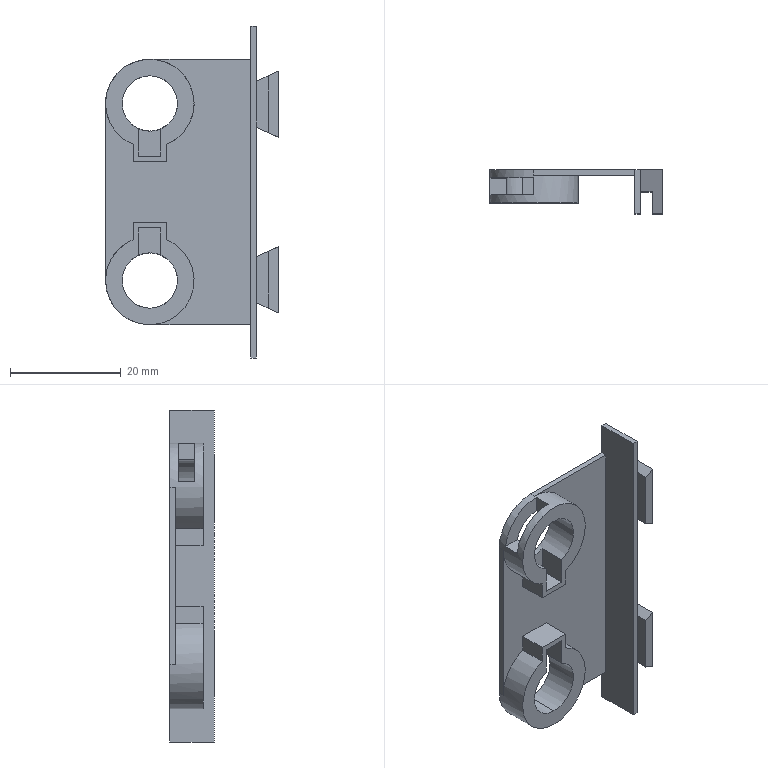Component | SolidWorks | DriveBracketBase-1 | 1 solid | 49 faces | box 31.25 x 8 x 60 mm | volume 3163 mm3 | plane 42 | cylinder 7 | commonest cylinder face diameters 10 x4 16 x3
build123d program:
from build123d import *

# Parameters (mm, degrees)
SKETCH1_W           = 60
SKETCH1_H           = 30
BOSS_EXTRUDE1_DEPTH = 1
BOSS_EXTRUDE2_DEPTH = 4
BOSS_EXTRUDE3_DEPTH = 4
SKETCH4_R           = 3
CUT_EXTRUDE1_DEPTH  = 4
SKETCH5_W           = 60
SKETCH5_H           = 36.5
BOSS_EXTRUDE4_DEPTH = 1
BOSS_EXTRUDE5_DEPTH = 5
CUT_EXTRUDE2_START  = -5
CUT_EXTRUDE2_DEPTH  = 5
SKETCH9_W           = 6.916
SKETCH9_H           = 3
CUT_EXTRUDE3_DEPTH  = 8
SKETCH10_W          = 60
SKETCH10_H          = 22
CUT_EXTRUDE4_DEPTH  = 8
CUT_EXTRUDE5_START  = -8
SKETCH11_R          = 5
CUT_EXTRUDE5_DEPTH  = 8
BOSS_EXTRUDE6_DEPTH = 4


with BuildPart() as part:
    # Sketch1 → Boss-Extrude1 (new body)
    with BuildSketch(Plane(origin=(0, 0, 0), x_dir=(1, 0, 0), z_dir=(0, 1, 0))):
        with Locations((30, 15)):
            Rectangle(SKETCH1_W, SKETCH1_H)
    extrude(amount=BOSS_EXTRUDE1_DEPTH)

    # Sketch2 → Boss-Extrude2 (add)
    with BuildSketch(Plane.XY):
        Polygon((10, 0), (8.135, -4), (20.135, -4), (18.27, 0), align=None)
        Polygon((50, 0), (51.865, -4), (39.865, -4), (41.73, 0), align=None)
    extrude(amount=-BOSS_EXTRUDE2_DEPTH)

    # Sketch3 → Boss-Extrude3 (add)
    with BuildSketch(Plane(origin=(0, 0, -30), x_dir=(-1, 0, 0), z_dir=(0, 0, -1))):
        Polygon((-50, 0), (-51.865, -4), (-58.135, -4), (-60, 0), align=None)
        Polygon((-41.73, 0), (-39.865, -4), (-20.135, -4), (-18.27, 0), align=None)
        Polygon((-10, 0), (-8.135, -4), (-1.865, -4), (0, 0), align=None)
    extrude(amount=-BOSS_EXTRUDE3_DEPTH)

    # Sketch4 → Cut-Extrude1 (cut)
    with BuildSketch(Plane(origin=(0, 1, 0), x_dir=(1, 0, 0), z_dir=(0, 1, 0))):
        with Locations(Location((6, 15, 0), (0, 0, 270))):
            Circle(SKETCH4_R)
        with Locations(Location((54, 15, 0), (0, 0, 90))):
            Circle(SKETCH4_R)
    extrude(amount=-CUT_EXTRUDE1_DEPTH, mode=Mode.SUBTRACT)

    # Sketch5 → Boss-Extrude4 (add)
    with BuildSketch(Plane.XY):
        with Locations((30, 19.25)):
            Rectangle(SKETCH5_W, SKETCH5_H)
    extrude(amount=-BOSS_EXTRUDE4_DEPTH)

    # Sketch6 → Boss-Extrude5 (add)
    # profile 1 of 2: a face of its own
    with BuildSketch(Plane(origin=(0, 0, -1), x_dir=(-1, 0, 0), z_dir=(0, 0, -1))):
        with BuildLine():
            Line((-35.5, 22.25), (-35.5, 16.25))
            Line((-35.5, 16.25), (-38.584, 16.25))
            ThreePointArc((-38.584, 16.25), (-54, 19.25), (-38.584, 22.25))
            Line((-38.584, 22.25), (-35.5, 22.25))
        make_face()
        with BuildLine():
            Line((-36.5, 21.25), (-36.5, 17.25))
            Line((-36.5, 17.25), (-41.417, 17.25))
            ThreePointArc((-41.417, 17.25), (-51, 19.25), (-41.417, 21.25))
            Line((-41.417, 21.25), (-36.5, 21.25))
        make_face(mode=Mode.SUBTRACT)
    # profile 2 of 2: a face of its own
    with BuildSketch(Plane(origin=(0, 0, -1), x_dir=(-1, 0, 0), z_dir=(0, 0, -1))):
        with BuildLine():
            Line((-24.5, 22.25), (-21.416, 22.25))
            ThreePointArc((-21.416, 22.25), (-6, 19.25), (-21.416, 16.25))
            Line((-21.416, 16.25), (-24.5, 16.25))
            Line((-24.5, 16.25), (-24.5, 22.25))
        make_face()
        with BuildLine():
            Line((-23.5, 21.25), (-23.5, 17.25))
            Line((-23.5, 17.25), (-18.583, 17.25))
            ThreePointArc((-18.583, 17.25), (-9, 19.25), (-18.583, 21.25))
            Line((-18.583, 21.25), (-23.5, 21.25))
        make_face(mode=Mode.SUBTRACT)
    extrude(amount=BOSS_EXTRUDE5_DEPTH)

    # Sketch8 → Cut-Extrude2 (cut)
    with BuildSketch(Plane(origin=(0, 0, -1), x_dir=(-1, 0, 0), z_dir=(0, 0, -1)).offset(CUT_EXTRUDE2_START)):
        with BuildLine():
            Line((-46, 27.25), (-14, 27.25))
            ThreePointArc((-14, 27.25), (-8.343, 24.907), (-6, 19.25))
            Line((-6, 19.25), (-6, 1))
            Line((-6, 1), (0, 1))
            Line((0, 1), (0, 37.5))
            Line((0, 37.5), (-60, 37.5))
            Line((-60, 37.5), (-60, 1))
            Line((-60, 1), (-54, 1))
            Line((-54, 1), (-54, 19.25))
            ThreePointArc((-54, 19.25), (-51.657, 24.907), (-46, 27.25))
        make_face()
    extrude(amount=CUT_EXTRUDE2_DEPTH, mode=Mode.SUBTRACT)

    # Sketch9 → Cut-Extrude3 (cut)
    with BuildSketch(Plane(origin=(0, 27.25, 0), x_dir=(1, 0, 0), z_dir=(0, 1, 0))):
        with Locations((9.458, 3)):
            Rectangle(SKETCH9_W, SKETCH9_H)
    extrude(amount=-CUT_EXTRUDE3_DEPTH, mode=Mode.SUBTRACT)

    # Sketch10 → Cut-Extrude4 (cut)
    with BuildSketch(Plane(origin=(0, 1, 0), x_dir=(1, 0, 0), z_dir=(0, 1, 0))):
        with Locations((30, 19)):
            Rectangle(SKETCH10_W, SKETCH10_H)
    extrude(amount=-CUT_EXTRUDE4_DEPTH, mode=Mode.SUBTRACT)

    # Sketch11 → Cut-Extrude5 (cut)
    with BuildSketch(Plane(origin=(0, 0, -1), x_dir=(-1, 0, 0), z_dir=(0, 0, -1)).offset(CUT_EXTRUDE5_START)):
        with Locations(Location((-46, 19.25, 0), (0, 0, 23.578))):
            Circle(SKETCH11_R)
        with Locations(Location((-14, 19.25, 0), (0, 0, 203.578))):
            Circle(SKETCH11_R)
    extrude(amount=CUT_EXTRUDE5_DEPTH, mode=Mode.SUBTRACT)

    # Sketch12 → Boss-Extrude6 (add)
    with BuildSketch(Plane(origin=(0, 0, -4), x_dir=(-1, 0, 0), z_dir=(0, 0, -1))):
        Polygon((-19.274, -2.154), (-20.135, -4), (-8.135, -4), (-8.995, -2.154), align=None)
        Polygon((-51.005, -2.154), (-51.865, -4), (-39.865, -4), (-40.726, -2.154), align=None)
    extrude(amount=BOSS_EXTRUDE6_DEPTH)


solid = part.part

# Placed as in the assembly
solid = solid.moved(Location((-45.793, 11.147, 946.064), (-90, 0, 90)))